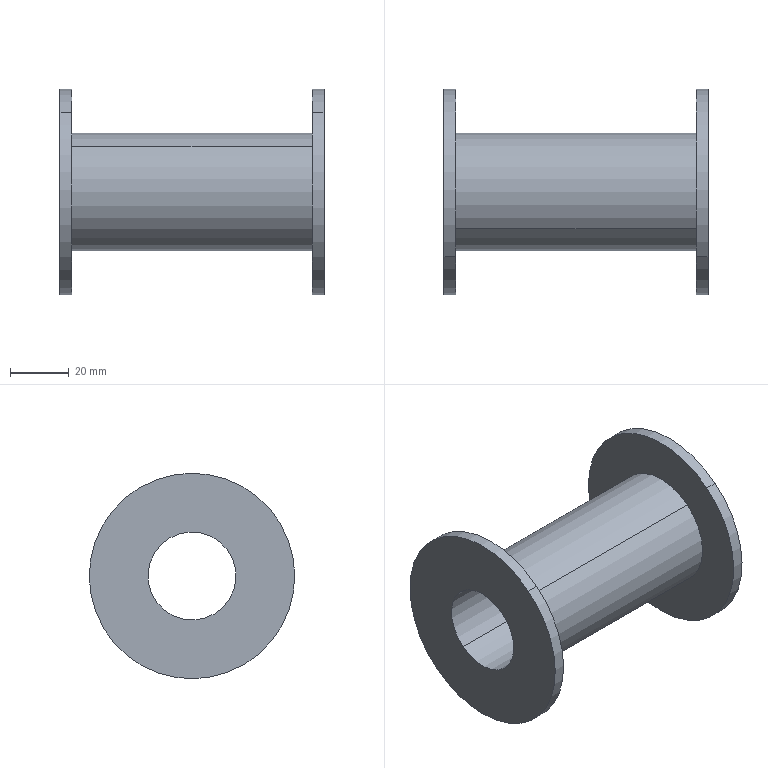Component | SolidWorks | Pulley-1 | 1 solid | 12 faces | box 90 x 70 x 70 mm | volume 70215 mm3 | cylinder 8 | plane 4 | commonest cylinder face diameters 70 x4 30 x2 40 x2
build123d program:
from build123d import *


with BuildPart() as part:
    # Sketch1 → Revolve1 (revolve)
    with BuildSketch(Plane.XY, mode=Mode.PRIVATE) as revolve1_sk:
        Polygon((0, 15), (0, 35), (4, 35), (4, 20), (86, 20), (86, 35), (90, 35), (90, 15), align=None)
    revolve(revolve1_sk.sketch.rotate(Axis((0, 0, 0), (1, 0, 0)), 90), axis=Axis((0, 0, 0), (1, 0, 0)))


solid = part.part

# Placed as in the assembly
solid = solid.moved(Location((730.2, -310.334, 1321.399), (0, 0, 0)))
STEP:
#1=COLOUR_RGB('',0.7922,0.8196,0.9333);
#2=FILL_AREA_STYLE_COLOUR('',#1);
#3=FILL_AREA_STYLE('',(#2));
#4=SURFACE_STYLE_FILL_AREA(#3);
#5=SURFACE_SIDE_STYLE('',(#4));
#6=SURFACE_STYLE_USAGE(.BOTH.,#5);
#7=PRESENTATION_STYLE_ASSIGNMENT((#6));
#8=CARTESIAN_POINT('',(32.291,-11.846,51.565));
#9=VERTEX_POINT('',#8);
#10=CARTESIAN_POINT('',(32.291,-12.59,52.482));
#11=VERTEX_POINT('',#10);
#12=CARTESIAN_POINT('',(32.291,-12.218,52.024));
#13=DIRECTION('',(-1.,0.,0.));
#14=DIRECTION('',(0.,-0.6297,0.7768));
#15=AXIS2_PLACEMENT_3D('',#12,#13,#14);
#16=CIRCLE('',#15,0.5906);
#17=EDGE_CURVE('',#9,#11,#16,.T.);
#18=ORIENTED_EDGE('',*,*,#17,.F.);
#19=CARTESIAN_POINT('',(28.748,-11.846,51.565));
#20=VERTEX_POINT('',#19);
#21=CARTESIAN_POINT('',(28.748,-11.846,51.565));
#22=DIRECTION('',(-1.,0.,0.));
#23=VECTOR('',#22,39.37);
#24=LINE('',#21,#23);
#25=EDGE_CURVE('',#9,#20,#24,.T.);
#26=ORIENTED_EDGE('',*,*,#25,.T.);
#27=CARTESIAN_POINT('',(28.748,-12.59,52.482));
#28=VERTEX_POINT('',#27);
#29=CARTESIAN_POINT('',(28.748,-12.218,52.024));
#30=DIRECTION('',(-1.,0.,0.));
#31=DIRECTION('',(0.,-0.6297,0.7768));
#32=AXIS2_PLACEMENT_3D('',#29,#30,#31);
#33=CIRCLE('',#32,0.5906);
#34=EDGE_CURVE('',#20,#28,#33,.T.);
#35=ORIENTED_EDGE('',*,*,#34,.T.);
#36=CARTESIAN_POINT('',(28.748,-12.59,52.482));
#37=DIRECTION('',(-1.,0.,0.));
#38=VECTOR('',#37,39.37);
#39=LINE('',#36,#38);
#40=EDGE_CURVE('',#11,#28,#39,.T.);
#41=ORIENTED_EDGE('',*,*,#40,.F.);
#42=EDGE_LOOP('',(#18,#26,#35,#41));
#43=FACE_OUTER_BOUND('',#42,.T.);
#44=CARTESIAN_POINT('',(28.748,-12.218,52.024));
#45=DIRECTION('',(-1.,0.,0.));
#46=DIRECTION('',(0.,-0.6297,0.7768));
#47=AXIS2_PLACEMENT_3D('',#44,#45,#46);
#48=CYLINDRICAL_SURFACE('',#47,0.5906);
#49=ADVANCED_FACE('',(#43),#48,.F.);
#50=CARTESIAN_POINT('',(32.291,-13.086,53.094));
#51=VERTEX_POINT('',#50);
#52=CARTESIAN_POINT('',(32.291,-11.35,50.953));
#53=VERTEX_POINT('',#52);
#54=CARTESIAN_POINT('',(32.291,-12.218,52.024));
#55=DIRECTION('',(-1.,0.,0.));
#56=DIRECTION('',(0.,-0.6297,0.7768));
#57=AXIS2_PLACEMENT_3D('',#54,#55,#56);
#58=CIRCLE('',#57,1.378);
#59=EDGE_CURVE('',#51,#53,#58,.T.);
#60=ORIENTED_EDGE('',*,*,#59,.T.);
#61=CARTESIAN_POINT('',(32.134,-11.35,50.953));
#62=VERTEX_POINT('',#61);
#63=CARTESIAN_POINT('',(28.748,-11.35,50.953));
#64=DIRECTION('',(-1.,0.,0.));
#65=VECTOR('',#64,39.37);
#66=LINE('',#63,#65);
#67=EDGE_CURVE('',#53,#62,#66,.T.);
#68=ORIENTED_EDGE('',*,*,#67,.T.);
#69=CARTESIAN_POINT('',(32.134,-13.086,53.094));
#70=VERTEX_POINT('',#69);
#71=CARTESIAN_POINT('',(32.134,-12.218,52.024));
#72=DIRECTION('',(-1.,0.,0.));
#73=DIRECTION('',(0.,-0.6297,0.7768));
#74=AXIS2_PLACEMENT_3D('',#71,#72,#73);
#75=CIRCLE('',#74,1.378);
#76=EDGE_CURVE('',#70,#62,#75,.T.);
#77=ORIENTED_EDGE('',*,*,#76,.F.);
#78=CARTESIAN_POINT('',(28.748,-13.086,53.094));
#79=DIRECTION('',(-1.,0.,0.));
#80=VECTOR('',#79,39.37);
#81=LINE('',#78,#80);
#82=EDGE_CURVE('',#51,#70,#81,.T.);
#83=ORIENTED_EDGE('',*,*,#82,.F.);
#84=EDGE_LOOP('',(#60,#68,#77,#83));
#85=FACE_OUTER_BOUND('',#84,.T.);
#86=CARTESIAN_POINT('',(28.748,-12.218,52.024));
#87=DIRECTION('',(-1.,0.,0.));
#88=DIRECTION('',(0.,-0.6297,0.7768));
#89=AXIS2_PLACEMENT_3D('',#86,#87,#88);
#90=CYLINDRICAL_SURFACE('',#89,1.378);
#91=ADVANCED_FACE('',(#85),#90,.T.);
#92=CARTESIAN_POINT('',(32.134,-12.714,52.635));
#93=VERTEX_POINT('',#92);
#94=CARTESIAN_POINT('',(32.134,-11.722,51.412));
#95=VERTEX_POINT('',#94);
#96=CARTESIAN_POINT('',(32.134,-12.218,52.024));
#97=DIRECTION('',(-1.,0.,0.));
#98=DIRECTION('',(0.,-0.6297,0.7768));
#99=AXIS2_PLACEMENT_3D('',#96,#97,#98);
#100=CIRCLE('',#99,0.7874);
#101=EDGE_CURVE('',#93,#95,#100,.T.);
#102=ORIENTED_EDGE('',*,*,#101,.T.);
#103=CARTESIAN_POINT('',(28.906,-11.722,51.412));
#104=VERTEX_POINT('',#103);
#105=CARTESIAN_POINT('',(28.748,-11.722,51.412));
#106=DIRECTION('',(-1.,0.,0.));
#107=VECTOR('',#106,39.37);
#108=LINE('',#105,#107);
#109=EDGE_CURVE('',#95,#104,#108,.T.);
#110=ORIENTED_EDGE('',*,*,#109,.T.);
#111=CARTESIAN_POINT('',(28.906,-12.714,52.635));
#112=VERTEX_POINT('',#111);
#113=CARTESIAN_POINT('',(28.906,-12.218,52.024));
#114=DIRECTION('',(-1.,0.,0.));
#115=DIRECTION('',(0.,-0.6297,0.7768));
#116=AXIS2_PLACEMENT_3D('',#113,#114,#115);
#117=CIRCLE('',#116,0.7874);
#118=EDGE_CURVE('',#112,#104,#117,.T.);
#119=ORIENTED_EDGE('',*,*,#118,.F.);
#120=CARTESIAN_POINT('',(28.748,-12.714,52.635));
#121=DIRECTION('',(-1.,0.,0.));
#122=VECTOR('',#121,39.37);
#123=LINE('',#120,#122);
#124=EDGE_CURVE('',#93,#112,#123,.T.);
#125=ORIENTED_EDGE('',*,*,#124,.F.);
#126=EDGE_LOOP('',(#102,#110,#119,#125));
#127=FACE_OUTER_BOUND('',#126,.T.);
#128=CARTESIAN_POINT('',(28.748,-12.218,52.024));
#129=DIRECTION('',(-1.,0.,0.));
#130=DIRECTION('',(0.,-0.6297,0.7768));
#131=AXIS2_PLACEMENT_3D('',#128,#129,#130);
#132=CYLINDRICAL_SURFACE('',#131,0.7874);
#133=ADVANCED_FACE('',(#127),#132,.T.);
#134=CARTESIAN_POINT('',(28.906,-13.086,53.094));
#135=VERTEX_POINT('',#134);
#136=CARTESIAN_POINT('',(28.906,-11.35,50.953));
#137=VERTEX_POINT('',#136);
#138=CARTESIAN_POINT('',(28.906,-12.218,52.024));
#139=DIRECTION('',(-1.,0.,0.));
#140=DIRECTION('',(0.,-0.6297,0.7768));
#141=AXIS2_PLACEMENT_3D('',#138,#139,#140);
#142=CIRCLE('',#141,1.378);
#143=EDGE_CURVE('',#135,#137,#142,.T.);
#144=ORIENTED_EDGE('',*,*,#143,.T.);
#145=CARTESIAN_POINT('',(28.748,-11.35,50.953));
#146=VERTEX_POINT('',#145);
#147=CARTESIAN_POINT('',(28.748,-11.35,50.953));
#148=DIRECTION('',(-1.,0.,0.));
#149=VECTOR('',#148,39.37);
#150=LINE('',#147,#149);
#151=EDGE_CURVE('',#137,#146,#150,.T.);
#152=ORIENTED_EDGE('',*,*,#151,.T.);
#153=CARTESIAN_POINT('',(28.748,-13.086,53.094));
#154=VERTEX_POINT('',#153);
#155=CARTESIAN_POINT('',(28.748,-12.218,52.024));
#156=DIRECTION('',(-1.,0.,0.));
#157=DIRECTION('',(0.,-0.6297,0.7768));
#158=AXIS2_PLACEMENT_3D('',#155,#156,#157);
#159=CIRCLE('',#158,1.378);
#160=EDGE_CURVE('',#154,#146,#159,.T.);
#161=ORIENTED_EDGE('',*,*,#160,.F.);
#162=CARTESIAN_POINT('',(28.748,-13.086,53.094));
#163=DIRECTION('',(-1.,0.,0.));
#164=VECTOR('',#163,39.37);
#165=LINE('',#162,#164);
#166=EDGE_CURVE('',#135,#154,#165,.T.);
#167=ORIENTED_EDGE('',*,*,#166,.F.);
#168=EDGE_LOOP('',(#144,#152,#161,#167));
#169=FACE_OUTER_BOUND('',#168,.T.);
#170=CARTESIAN_POINT('',(28.748,-12.218,52.024));
#171=DIRECTION('',(-1.,0.,0.));
#172=DIRECTION('',(0.,-0.6297,0.7768));
#173=AXIS2_PLACEMENT_3D('',#170,#171,#172);
#174=CYLINDRICAL_SURFACE('',#173,1.378);
#175=ADVANCED_FACE('',(#169),#174,.T.);
#176=ORIENTED_EDGE('',*,*,#151,.F.);
#177=CARTESIAN_POINT('',(28.906,-12.218,52.024));
#178=DIRECTION('',(-1.,0.,0.));
#179=DIRECTION('',(0.,-0.6297,0.7768));
#180=AXIS2_PLACEMENT_3D('',#177,#178,#179);
#181=CIRCLE('',#180,1.378);
#182=EDGE_CURVE('',#137,#135,#181,.T.);
#183=ORIENTED_EDGE('',*,*,#182,.T.);
#184=ORIENTED_EDGE('',*,*,#166,.T.);
#185=CARTESIAN_POINT('',(28.748,-12.218,52.024));
#186=DIRECTION('',(-1.,0.,0.));
#187=DIRECTION('',(0.,-0.6297,0.7768));
#188=AXIS2_PLACEMENT_3D('',#185,#186,#187);
#189=CIRCLE('',#188,1.378);
#190=EDGE_CURVE('',#146,#154,#189,.T.);
#191=ORIENTED_EDGE('',*,*,#190,.F.);
#192=EDGE_LOOP('',(#176,#183,#184,#191));
#193=FACE_OUTER_BOUND('',#192,.T.);
#194=CARTESIAN_POINT('',(28.748,-12.218,52.024));
#195=DIRECTION('',(-1.,0.,0.));
#196=DIRECTION('',(0.,-0.6297,0.7768));
#197=AXIS2_PLACEMENT_3D('',#194,#195,#196);
#198=CYLINDRICAL_SURFACE('',#197,1.378);
#199=ADVANCED_FACE('',(#193),#198,.T.);
#200=ORIENTED_EDGE('',*,*,#143,.F.);
#201=ORIENTED_EDGE('',*,*,#182,.F.);
#202=EDGE_LOOP('',(#200,#201));
#203=FACE_OUTER_BOUND('',#202,.T.);
#204=ORIENTED_EDGE('',*,*,#118,.T.);
#205=CARTESIAN_POINT('',(28.906,-12.218,52.024));
#206=DIRECTION('',(-1.,0.,0.));
#207=DIRECTION('',(0.,-0.6297,0.7768));
#208=AXIS2_PLACEMENT_3D('',#205,#206,#207);
#209=CIRCLE('',#208,0.7874);
#210=EDGE_CURVE('',#104,#112,#209,.T.);
#211=ORIENTED_EDGE('',*,*,#210,.T.);
#212=EDGE_LOOP('',(#204,#211));
#213=FACE_BOUND('',#212,.T.);
#214=CARTESIAN_POINT('',(28.906,-11.147,52.891));
#215=DIRECTION('',(-1.,0.,0.));
#216=DIRECTION('',(0.,-0.6297,0.7768));
#217=AXIS2_PLACEMENT_3D('',#214,#215,#216);
#218=PLANE('',#217);
#219=ADVANCED_FACE('',(#203,#213),#218,.F.);
#220=ORIENTED_EDGE('',*,*,#109,.F.);
#221=CARTESIAN_POINT('',(32.134,-12.218,52.024));
#222=DIRECTION('',(-1.,0.,0.));
#223=DIRECTION('',(0.,-0.6297,0.7768));
#224=AXIS2_PLACEMENT_3D('',#221,#222,#223);
#225=CIRCLE('',#224,0.7874);
#226=EDGE_CURVE('',#95,#93,#225,.T.);
#227=ORIENTED_EDGE('',*,*,#226,.T.);
#228=ORIENTED_EDGE('',*,*,#124,.T.);
#229=ORIENTED_EDGE('',*,*,#210,.F.);
#230=EDGE_LOOP('',(#220,#227,#228,#229));
#231=FACE_OUTER_BOUND('',#230,.T.);
#232=CARTESIAN_POINT('',(28.748,-12.218,52.024));
#233=DIRECTION('',(-1.,0.,0.));
#234=DIRECTION('',(0.,-0.6297,0.7768));
#235=AXIS2_PLACEMENT_3D('',#232,#233,#234);
#236=CYLINDRICAL_SURFACE('',#235,0.7874);
#237=ADVANCED_FACE('',(#231),#236,.T.);
#238=ORIENTED_EDGE('',*,*,#101,.F.);
#239=ORIENTED_EDGE('',*,*,#226,.F.);
#240=EDGE_LOOP('',(#238,#239));
#241=FACE_BOUND('',#240,.T.);
#242=ORIENTED_EDGE('',*,*,#76,.T.);
#243=CARTESIAN_POINT('',(32.134,-12.218,52.024));
#244=DIRECTION('',(-1.,0.,0.));
#245=DIRECTION('',(0.,-0.6297,0.7768));
#246=AXIS2_PLACEMENT_3D('',#243,#244,#245);
#247=CIRCLE('',#246,1.378);
#248=EDGE_CURVE('',#62,#70,#247,.T.);
#249=ORIENTED_EDGE('',*,*,#248,.T.);
#250=EDGE_LOOP('',(#242,#249));
#251=FACE_OUTER_BOUND('',#250,.T.);
#252=CARTESIAN_POINT('',(32.134,-11.606,52.519));
#253=DIRECTION('',(1.,0.,0.));
#254=DIRECTION('',(0.,0.6297,-0.7768));
#255=AXIS2_PLACEMENT_3D('',#252,#253,#254);
#256=PLANE('',#255);
#257=ADVANCED_FACE('',(#241,#251),#256,.F.);
#258=ORIENTED_EDGE('',*,*,#67,.F.);
#259=CARTESIAN_POINT('',(32.291,-12.218,52.024));
#260=DIRECTION('',(-1.,0.,0.));
#261=DIRECTION('',(0.,-0.6297,0.7768));
#262=AXIS2_PLACEMENT_3D('',#259,#260,#261);
#263=CIRCLE('',#262,1.378);
#264=EDGE_CURVE('',#53,#51,#263,.T.);
#265=ORIENTED_EDGE('',*,*,#264,.T.);
#266=ORIENTED_EDGE('',*,*,#82,.T.);
#267=ORIENTED_EDGE('',*,*,#248,.F.);
#268=EDGE_LOOP('',(#258,#265,#266,#267));
#269=FACE_OUTER_BOUND('',#268,.T.);
#270=CARTESIAN_POINT('',(28.748,-12.218,52.024));
#271=DIRECTION('',(-1.,0.,0.));
#272=DIRECTION('',(0.,-0.6297,0.7768));
#273=AXIS2_PLACEMENT_3D('',#270,#271,#272);
#274=CYLINDRICAL_SURFACE('',#273,1.378);
#275=ADVANCED_FACE('',(#269),#274,.T.);
#276=ORIENTED_EDGE('',*,*,#59,.F.);
#277=ORIENTED_EDGE('',*,*,#264,.F.);
#278=EDGE_LOOP('',(#276,#277));
#279=FACE_OUTER_BOUND('',#278,.T.);
#280=CARTESIAN_POINT('',(32.291,-12.218,52.024));
#281=DIRECTION('',(-1.,0.,0.));
#282=DIRECTION('',(0.,-0.6297,0.7768));
#283=AXIS2_PLACEMENT_3D('',#280,#281,#282);
#284=CIRCLE('',#283,0.5906);
#285=EDGE_CURVE('',#11,#9,#284,.T.);
#286=ORIENTED_EDGE('',*,*,#285,.T.);
#287=ORIENTED_EDGE('',*,*,#17,.T.);
#288=EDGE_LOOP('',(#286,#287));
#289=FACE_BOUND('',#288,.T.);
#290=CARTESIAN_POINT('',(32.291,-11.147,52.891));
#291=DIRECTION('',(-1.,0.,0.));
#292=DIRECTION('',(0.,-0.6297,0.7768));
#293=AXIS2_PLACEMENT_3D('',#290,#291,#292);
#294=PLANE('',#293);
#295=ADVANCED_FACE('',(#279,#289),#294,.F.);
#296=ORIENTED_EDGE('',*,*,#25,.F.);
#297=ORIENTED_EDGE('',*,*,#285,.F.);
#298=ORIENTED_EDGE('',*,*,#40,.T.);
#299=CARTESIAN_POINT('',(28.748,-12.218,52.024));
#300=DIRECTION('',(-1.,0.,0.));
#301=DIRECTION('',(0.,-0.6297,0.7768));
#302=AXIS2_PLACEMENT_3D('',#299,#300,#301);
#303=CIRCLE('',#302,0.5906);
#304=EDGE_CURVE('',#28,#20,#303,.T.);
#305=ORIENTED_EDGE('',*,*,#304,.T.);
#306=EDGE_LOOP('',(#296,#297,#298,#305));
#307=FACE_OUTER_BOUND('',#306,.T.);
#308=CARTESIAN_POINT('',(28.748,-12.218,52.024));
#309=DIRECTION('',(-1.,0.,0.));
#310=DIRECTION('',(0.,-0.6297,0.7768));
#311=AXIS2_PLACEMENT_3D('',#308,#309,#310);
#312=CYLINDRICAL_SURFACE('',#311,0.5906);
#313=ADVANCED_FACE('',(#307),#312,.F.);
#314=ORIENTED_EDGE('',*,*,#304,.F.);
#315=ORIENTED_EDGE('',*,*,#34,.F.);
#316=EDGE_LOOP('',(#314,#315));
#317=FACE_BOUND('',#316,.T.);
#318=ORIENTED_EDGE('',*,*,#160,.T.);
#319=ORIENTED_EDGE('',*,*,#190,.T.);
#320=EDGE_LOOP('',(#318,#319));
#321=FACE_OUTER_BOUND('',#320,.T.);
#322=CARTESIAN_POINT('',(28.748,-11.759,52.395));
#323=DIRECTION('',(1.,0.,0.));
#324=DIRECTION('',(0.,0.6297,-0.7768));
#325=AXIS2_PLACEMENT_3D('',#322,#323,#324);
#326=PLANE('',#325);
#327=ADVANCED_FACE('',(#317,#321),#326,.F.);
#328=CLOSED_SHELL('',(#49,#91,#133,#175,#199,#219,#237,#257,#275,#295,#313,#327));
#329=MANIFOLD_SOLID_BREP('',#328);
#330=STYLED_ITEM('',(#7),#329);
#331=PRESENTATION_LAYER_ASSIGNMENT('','',(#330));
#332=CARTESIAN_POINT('',(0.,0.,0.));
#333=DIRECTION('',(0.,0.,1.));
#334=DIRECTION('',(1.,0.,0.));
#335=AXIS2_PLACEMENT_3D('',#332,#333,#334);
#336=(LENGTH_UNIT()NAMED_UNIT(*)SI_UNIT($,.METRE.));
#337=LENGTH_MEASURE_WITH_UNIT(LENGTH_MEASURE(0.0254),#336);
#338=DIMENSIONAL_EXPONENTS(1.,0.,0.,0.,0.,0.,0.);
#339=(CONVERSION_BASED_UNIT('',#337)LENGTH_UNIT()NAMED_UNIT(#338));
#340=UNCERTAINTY_MEASURE_WITH_UNIT(LENGTH_MEASURE(0.00001),#339,'','');
#341=(NAMED_UNIT(*)PLANE_ANGLE_UNIT()SI_UNIT($,.RADIAN.));
#342=(NAMED_UNIT(*)SI_UNIT($,.STERADIAN.)SOLID_ANGLE_UNIT());
#343=(GEOMETRIC_REPRESENTATION_CONTEXT(3)GLOBAL_UNCERTAINTY_ASSIGNED_CONTEXT((#340))GLOBAL_UNIT_ASSIGNED_CONTEXT((#339,#341,#342))REPRESENTATION_CONTEXT('',''));
#344=ADVANCED_BREP_SHAPE_REPRESENTATION('',(#329,#335),#343);
#345=(LENGTH_UNIT()NAMED_UNIT(*)SI_UNIT($,.METRE.));
#346=LENGTH_MEASURE_WITH_UNIT(LENGTH_MEASURE(0.0254),#345);
#347=DIMENSIONAL_EXPONENTS(1.,0.,0.,0.,0.,0.,0.);
#348=(CONVERSION_BASED_UNIT('',#346)LENGTH_UNIT()NAMED_UNIT(#347));
#349=UNCERTAINTY_MEASURE_WITH_UNIT(LENGTH_MEASURE(0.00001),#348,'','');
#350=(NAMED_UNIT(*)PLANE_ANGLE_UNIT()SI_UNIT($,.RADIAN.));
#351=(NAMED_UNIT(*)SI_UNIT($,.STERADIAN.)SOLID_ANGLE_UNIT());
#352=(GEOMETRIC_REPRESENTATION_CONTEXT(3)GLOBAL_UNCERTAINTY_ASSIGNED_CONTEXT((#349))GLOBAL_UNIT_ASSIGNED_CONTEXT((#348,#350,#351))REPRESENTATION_CONTEXT('',''));
#353=MECHANICAL_DESIGN_GEOMETRIC_PRESENTATION_REPRESENTATION('',(#330),#352);